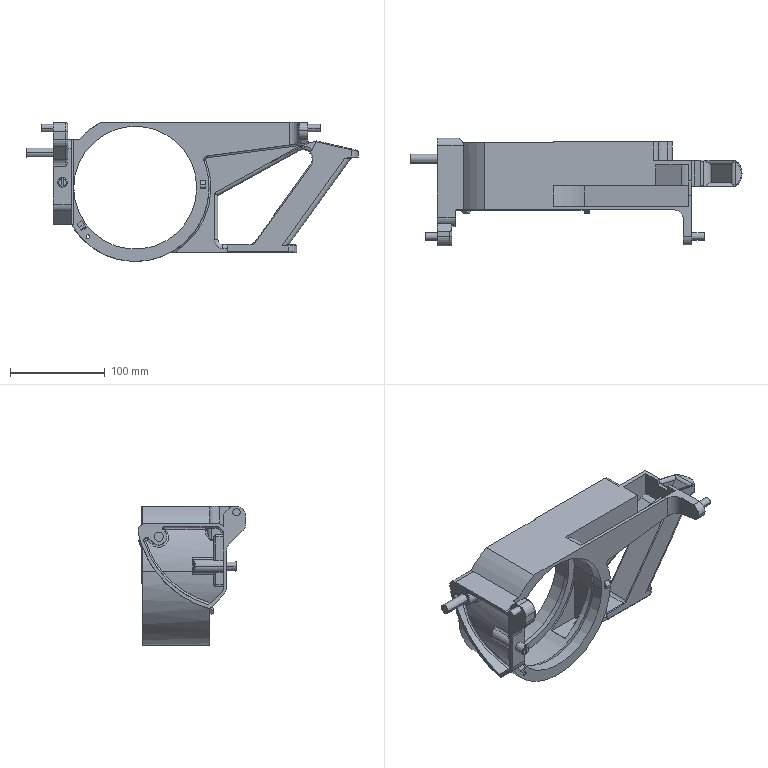Component | SolidWorks | Top base-1 | 1 solid | 332 faces | box 351 x 113.79 x 147 mm | volume 503823 mm3 | cylinder 148 | plane 128 | torus 26 | spline 18 | cone 8 | sphere 4 | commonest cylinder face diameters 4 x39 2 x16 8 x13 10 x13 156 x11 20 x9 6 x6 3.5 x4